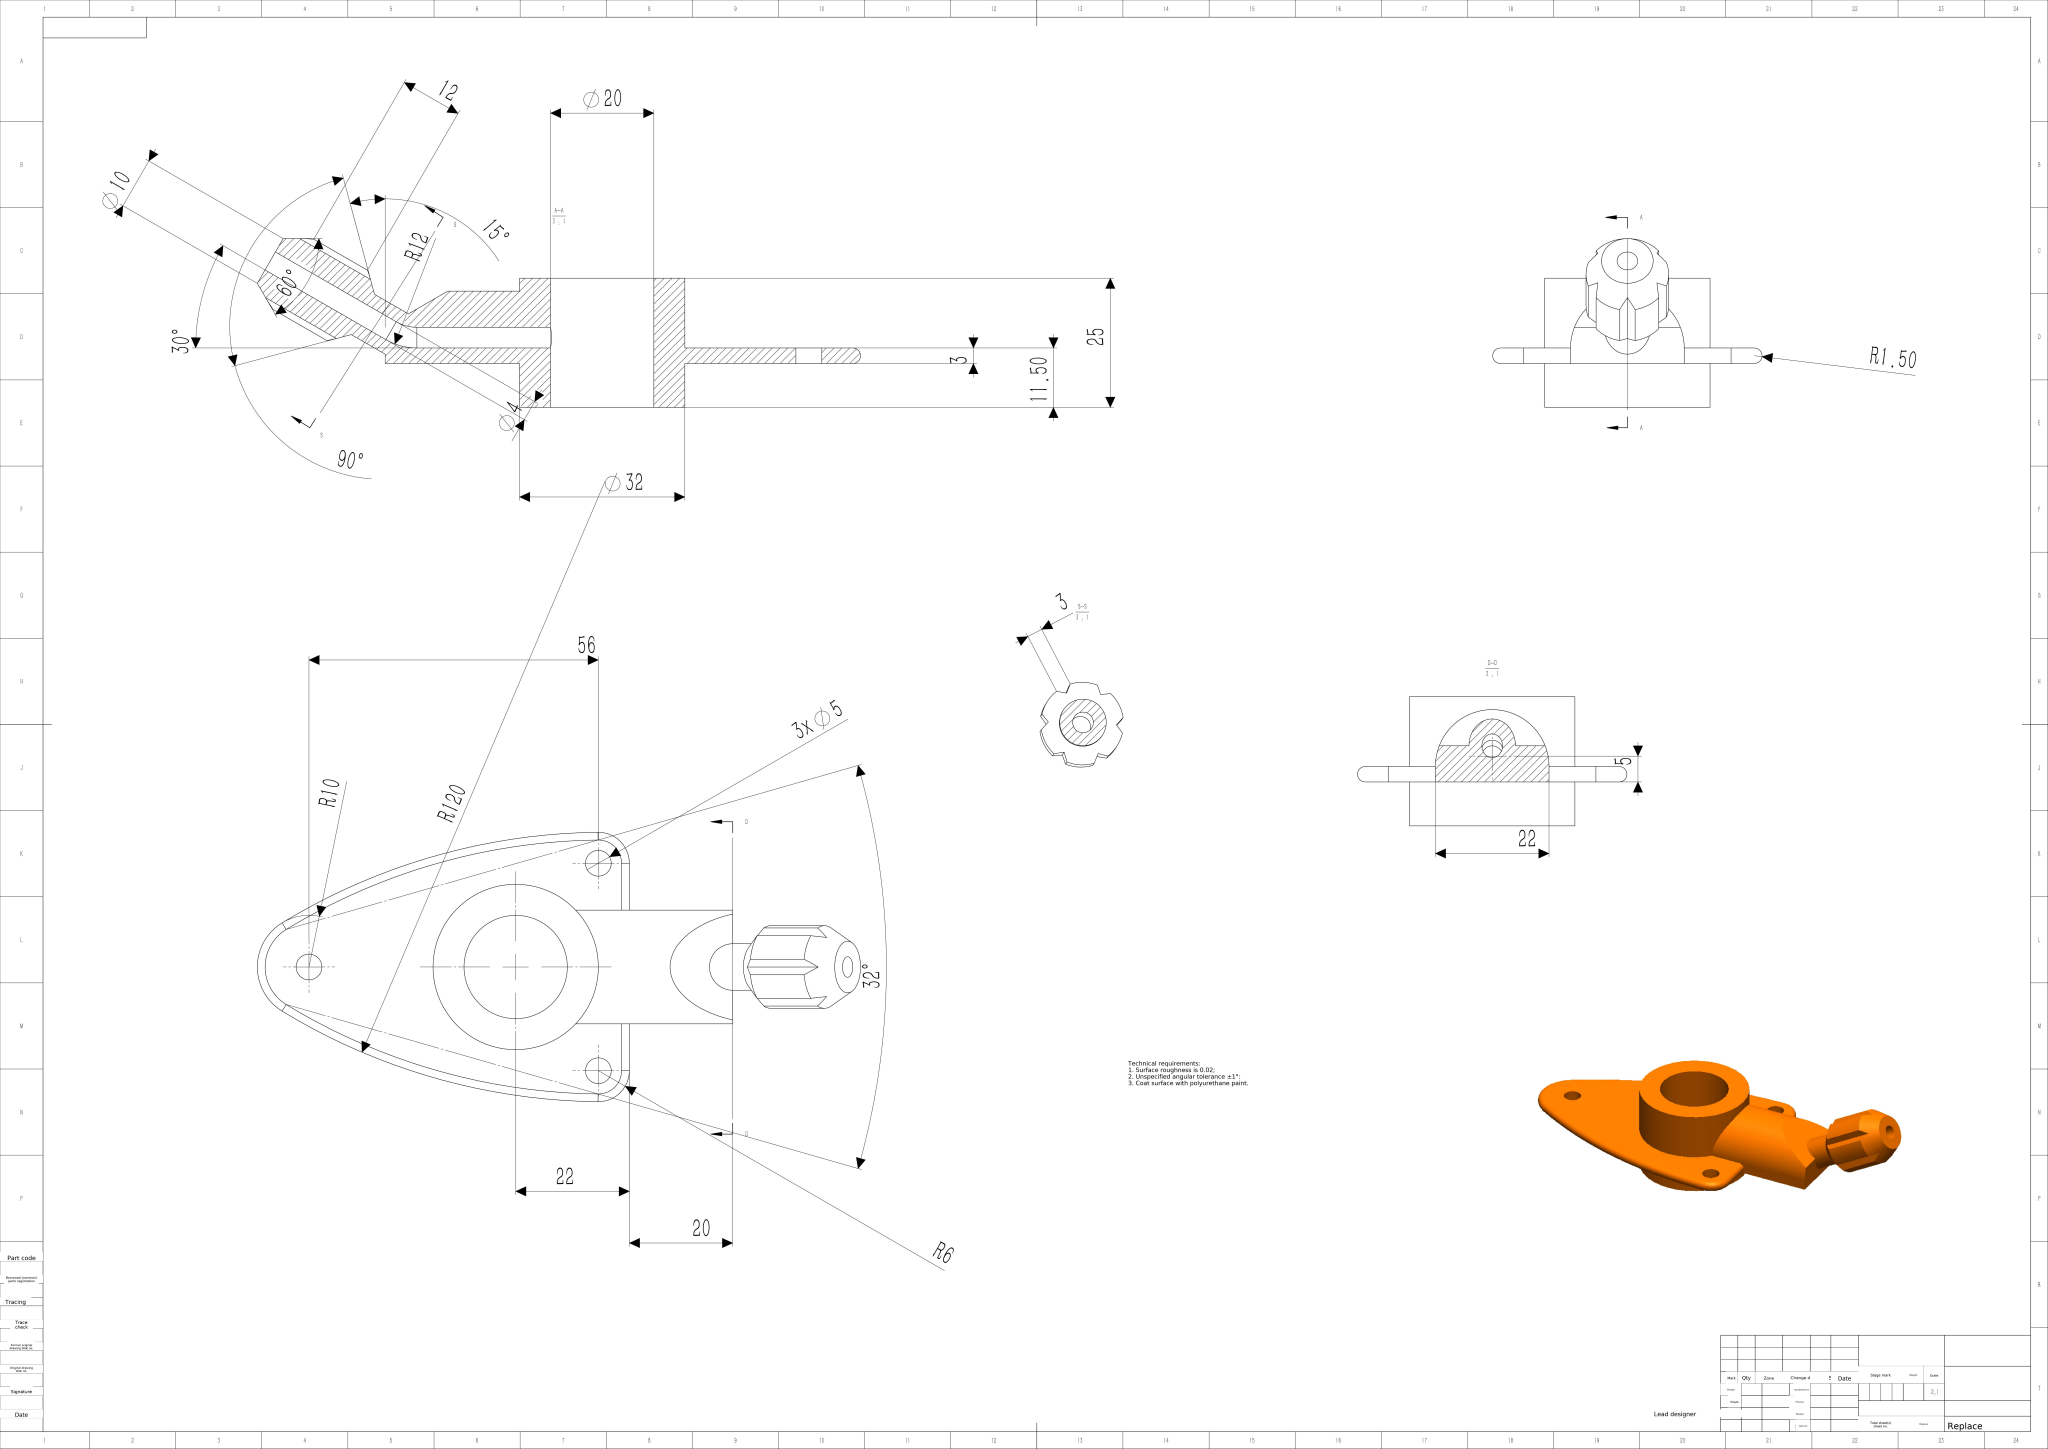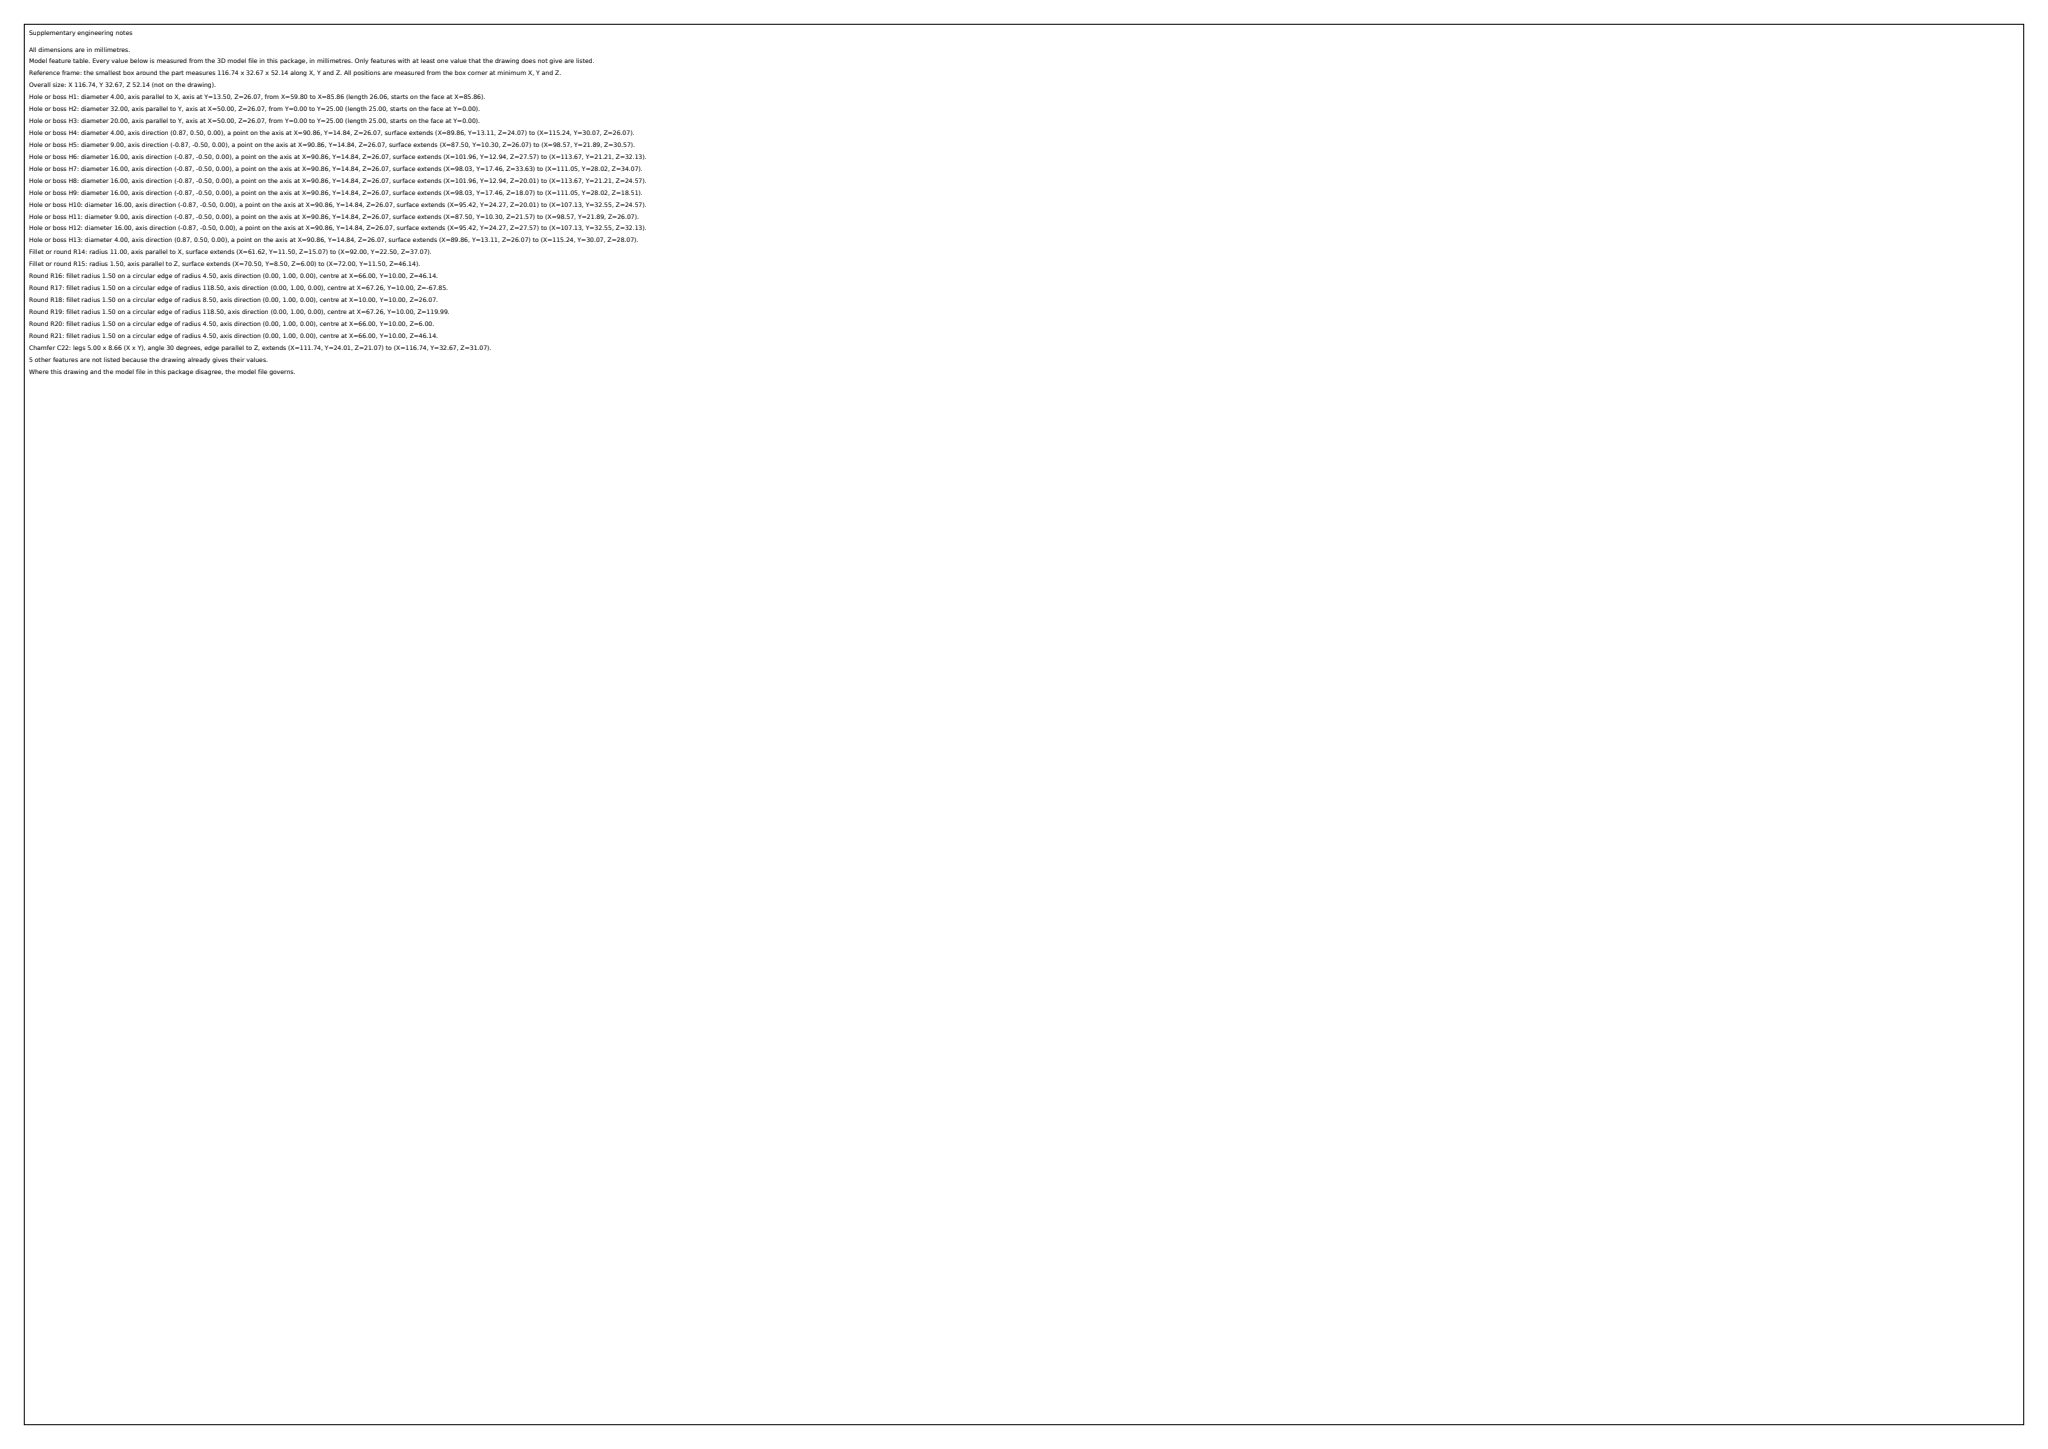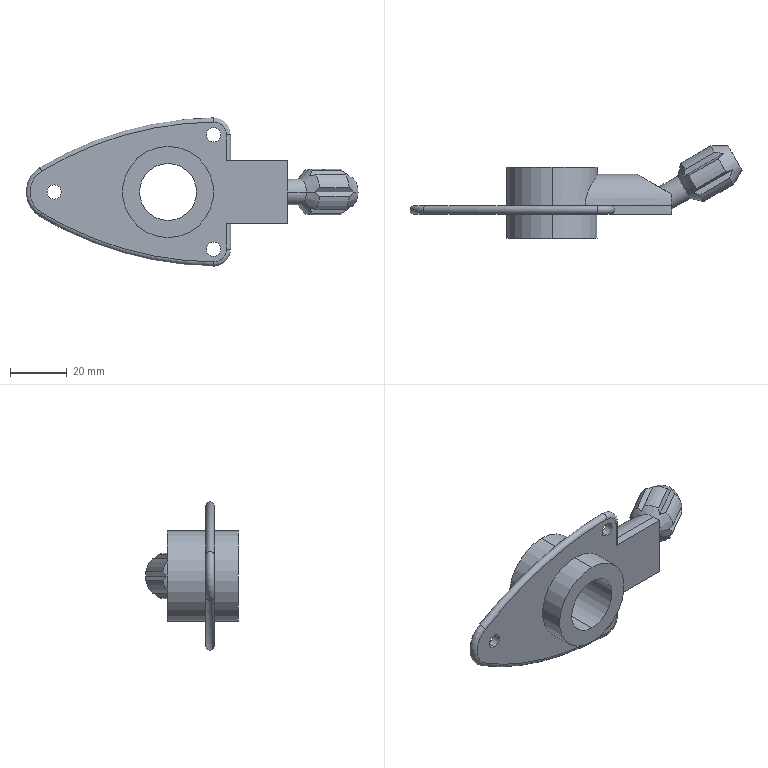Part | SolidWorks | mm | 1 solid | 60 faces | box 116.74 x 32.67 x 52.14 mm | volume 26975 mm3 | cylinder 27 | plane 21 | torus 8 | cone 4 | commonest cylinder face diameters 5 x6 16 x6 4 x4 32 x4 9 x2 20 x2 3 x2 22 x1